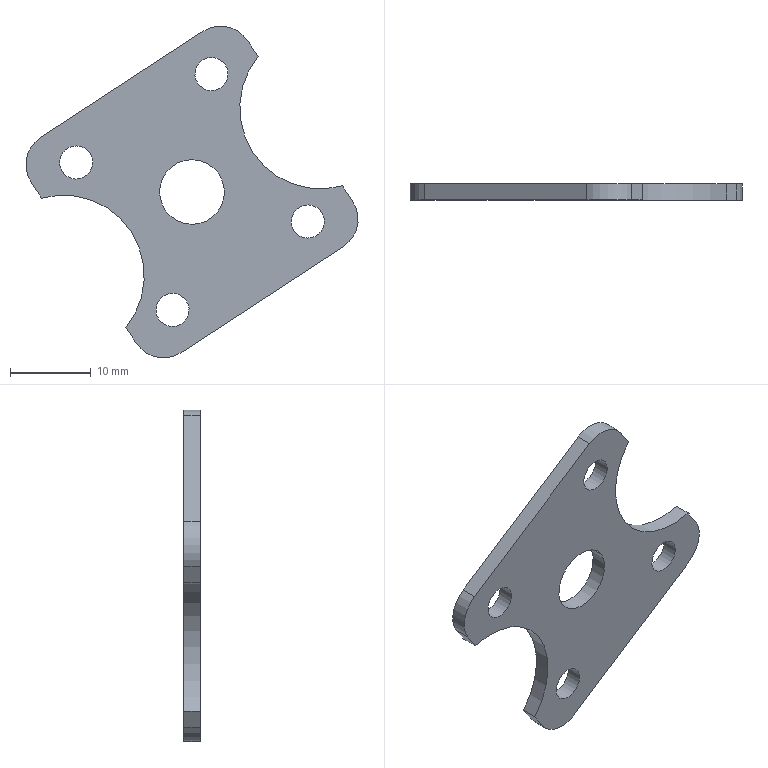Component | SolidWorks | FrontWheelSidePadPlate-1 | 1 solid | 25 faces | box 41.11 x 2 x 41.05 mm | volume 1410 mm3 | cylinder 17 | plane 8 | commonest cylinder face diameters 4.1 x8 8 x6 20 x3
build123d program:
from build123d import *

# Parameters (mm, degrees)
SKETCH1_R           = 2.05
SKETCH1_R_2         = 4
BOSS_EXTRUDE1_DEPTH = 2
FILLET1_R           = 4


with BuildPart() as part:
    # Sketch1 → Boss-Extrude1 (new body)
    with BuildSketch(Plane.XY):
        with BuildLine():
            Line((-16, -9.539), (-16, -15.9))
            Line((-16, -15.9), (16, -15.9))
            Line((16, -15.9), (16, -9.539))
            ThreePointArc((16, -9.539), (9, 0), (16, 9.539))
            Line((16, 9.539), (16, 15.9))
            Line((16, 15.9), (-16, 15.9))
            Line((-16, 15.9), (-16, 9.539))
            ThreePointArc((-16, 9.539), (-10.938, 5.916), (-9, 0))
            ThreePointArc((-9, 0), (-10.938, -5.916), (-16, -9.539))
        make_face()
        with Locations((-10, -10.9)):
            Circle(SKETCH1_R, mode=Mode.SUBTRACT)
        with Locations((10, -10.9)):
            Circle(SKETCH1_R, mode=Mode.SUBTRACT)
        with Locations((-10, 10.9)):
            Circle(SKETCH1_R, mode=Mode.SUBTRACT)
        Circle(SKETCH1_R_2, mode=Mode.SUBTRACT)
        with Locations((10, 10.9)):
            Circle(SKETCH1_R, mode=Mode.SUBTRACT)
    extrude(amount=BOSS_EXTRUDE1_DEPTH)

    # Fillet1
    fillet1_edges = [part.edges().sort_by_distance(p)[0] for p in [
        (-16, 15.9, 1),
        (16, 15.9, 1),
        (16, -15.9, 1),
        (-16, -15.9, 1),
    ]]
    fillet(fillet1_edges, radius=FILLET1_R)


solid = part.part

# Placed as in the assembly
solid = solid.moved(Location((0.3183, 28.4, 37), (90, 0, 33.158)))
STEP:
#1=CARTESIAN_POINT('',(0.175,1.118,2.075));
#2=VERTEX_POINT('',#1);
#3=CARTESIAN_POINT('',(0.03985,1.118,1.987));
#4=VERTEX_POINT('',#3);
#5=CARTESIAN_POINT('',(0.1074,1.118,2.031));
#6=DIRECTION('',(0.,-1.,0.));
#7=DIRECTION('',(0.8372,0.,0.5469));
#8=AXIS2_PLACEMENT_3D('',#5,#6,#7);
#9=CIRCLE('',#8,0.08071);
#10=EDGE_CURVE('',#2,#4,#9,.T.);
#11=ORIENTED_EDGE('',*,*,#10,.F.);
#12=CARTESIAN_POINT('',(0.175,1.039,2.075));
#13=VERTEX_POINT('',#12);
#14=CARTESIAN_POINT('',(0.175,1.118,2.075));
#15=DIRECTION('',(0.,-1.,0.));
#16=VECTOR('',#15,39.37);
#17=LINE('',#14,#16);
#18=EDGE_CURVE('',#2,#13,#17,.T.);
#19=ORIENTED_EDGE('',*,*,#18,.T.);
#20=CARTESIAN_POINT('',(0.03985,1.039,1.987));
#21=VERTEX_POINT('',#20);
#22=CARTESIAN_POINT('',(0.1074,1.039,2.031));
#23=DIRECTION('',(0.,-1.,0.));
#24=DIRECTION('',(0.8372,0.,0.5469));
#25=AXIS2_PLACEMENT_3D('',#22,#23,#24);
#26=CIRCLE('',#25,0.08071);
#27=EDGE_CURVE('',#13,#21,#26,.T.);
#28=ORIENTED_EDGE('',*,*,#27,.T.);
#29=CARTESIAN_POINT('',(0.03985,1.118,1.987));
#30=DIRECTION('',(0.,-1.,0.));
#31=VECTOR('',#30,39.37);
#32=LINE('',#29,#31);
#33=EDGE_CURVE('',#4,#21,#32,.T.);
#34=ORIENTED_EDGE('',*,*,#33,.F.);
#35=EDGE_LOOP('',(#11,#19,#28,#34));
#36=FACE_OUTER_BOUND('',#35,.T.);
#37=CARTESIAN_POINT('',(0.1074,1.118,2.031));
#38=DIRECTION('',(0.,-1.,0.));
#39=DIRECTION('',(-0.8372,0.,-0.5469));
#40=AXIS2_PLACEMENT_3D('',#37,#38,#39);
#41=CYLINDRICAL_SURFACE('',#40,0.08071);
#42=ADVANCED_FACE('',(#36),#41,.F.);
#43=CARTESIAN_POINT('',(0.5093,1.118,1.269));
#44=VERTEX_POINT('',#43);
#45=CARTESIAN_POINT('',(0.6444,1.118,1.357));
#46=VERTEX_POINT('',#45);
#47=CARTESIAN_POINT('',(0.5768,1.118,1.313));
#48=DIRECTION('',(0.,1.,0.));
#49=DIRECTION('',(0.8372,0.,0.5469));
#50=AXIS2_PLACEMENT_3D('',#47,#48,#49);
#51=CIRCLE('',#50,0.08071);
#52=EDGE_CURVE('',#44,#46,#51,.T.);
#53=ORIENTED_EDGE('',*,*,#52,.T.);
#54=CARTESIAN_POINT('',(0.6444,1.039,1.357));
#55=VERTEX_POINT('',#54);
#56=CARTESIAN_POINT('',(0.6444,1.118,1.357));
#57=DIRECTION('',(0.,-1.,0.));
#58=VECTOR('',#57,39.37);
#59=LINE('',#56,#58);
#60=EDGE_CURVE('',#46,#55,#59,.T.);
#61=ORIENTED_EDGE('',*,*,#60,.T.);
#62=CARTESIAN_POINT('',(0.5093,1.039,1.269));
#63=VERTEX_POINT('',#62);
#64=CARTESIAN_POINT('',(0.5768,1.039,1.313));
#65=DIRECTION('',(0.,1.,0.));
#66=DIRECTION('',(0.8372,0.,0.5469));
#67=AXIS2_PLACEMENT_3D('',#64,#65,#66);
#68=CIRCLE('',#67,0.08071);
#69=EDGE_CURVE('',#63,#55,#68,.T.);
#70=ORIENTED_EDGE('',*,*,#69,.F.);
#71=CARTESIAN_POINT('',(0.5093,1.118,1.269));
#72=DIRECTION('',(0.,-1.,0.));
#73=VECTOR('',#72,39.37);
#74=LINE('',#71,#73);
#75=EDGE_CURVE('',#44,#63,#74,.T.);
#76=ORIENTED_EDGE('',*,*,#75,.F.);
#77=EDGE_LOOP('',(#53,#61,#70,#76));
#78=FACE_OUTER_BOUND('',#77,.T.);
#79=CARTESIAN_POINT('',(0.5768,1.118,1.313));
#80=DIRECTION('',(0.,-1.,0.));
#81=DIRECTION('',(-0.8372,0.,-0.5469));
#82=AXIS2_PLACEMENT_3D('',#79,#80,#81);
#83=CYLINDRICAL_SURFACE('',#82,0.08071);
#84=ADVANCED_FACE('',(#78),#83,.F.);
#85=CARTESIAN_POINT('',(-0.1499,1.118,0.838));
#86=VERTEX_POINT('',#85);
#87=CARTESIAN_POINT('',(-0.01478,1.118,0.9262));
#88=VERTEX_POINT('',#87);
#89=CARTESIAN_POINT('',(-0.08235,1.118,0.8821));
#90=DIRECTION('',(0.,1.,0.));
#91=DIRECTION('',(0.8372,0.,0.5469));
#92=AXIS2_PLACEMENT_3D('',#89,#90,#91);
#93=CIRCLE('',#92,0.08071);
#94=EDGE_CURVE('',#86,#88,#93,.T.);
#95=ORIENTED_EDGE('',*,*,#94,.T.);
#96=CARTESIAN_POINT('',(-0.01478,1.039,0.9262));
#97=VERTEX_POINT('',#96);
#98=CARTESIAN_POINT('',(-0.01478,1.118,0.9262));
#99=DIRECTION('',(0.,-1.,0.));
#100=VECTOR('',#99,39.37);
#101=LINE('',#98,#100);
#102=EDGE_CURVE('',#88,#97,#101,.T.);
#103=ORIENTED_EDGE('',*,*,#102,.T.);
#104=CARTESIAN_POINT('',(-0.1499,1.039,0.838));
#105=VERTEX_POINT('',#104);
#106=CARTESIAN_POINT('',(-0.08235,1.039,0.8821));
#107=DIRECTION('',(0.,1.,0.));
#108=DIRECTION('',(0.8372,0.,0.5469));
#109=AXIS2_PLACEMENT_3D('',#106,#107,#108);
#110=CIRCLE('',#109,0.08071);
#111=EDGE_CURVE('',#105,#97,#110,.T.);
#112=ORIENTED_EDGE('',*,*,#111,.F.);
#113=CARTESIAN_POINT('',(-0.1499,1.118,0.838));
#114=DIRECTION('',(0.,-1.,0.));
#115=VECTOR('',#114,39.37);
#116=LINE('',#113,#115);
#117=EDGE_CURVE('',#86,#105,#116,.T.);
#118=ORIENTED_EDGE('',*,*,#117,.F.);
#119=EDGE_LOOP('',(#95,#103,#112,#118));
#120=FACE_OUTER_BOUND('',#119,.T.);
#121=CARTESIAN_POINT('',(-0.08235,1.118,0.8821));
#122=DIRECTION('',(0.,-1.,0.));
#123=DIRECTION('',(-0.8372,0.,-0.5469));
#124=AXIS2_PLACEMENT_3D('',#121,#122,#123);
#125=CYLINDRICAL_SURFACE('',#124,0.08071);
#126=ADVANCED_FACE('',(#120),#125,.F.);
#127=CARTESIAN_POINT('',(-0.4842,1.118,1.645));
#128=VERTEX_POINT('',#127);
#129=CARTESIAN_POINT('',(-0.6193,1.118,1.556));
#130=VERTEX_POINT('',#129);
#131=CARTESIAN_POINT('',(-0.5518,1.118,1.601));
#132=DIRECTION('',(0.,-1.,0.));
#133=DIRECTION('',(0.8372,0.,0.5469));
#134=AXIS2_PLACEMENT_3D('',#131,#132,#133);
#135=CIRCLE('',#134,0.08071);
#136=EDGE_CURVE('',#128,#130,#135,.T.);
#137=ORIENTED_EDGE('',*,*,#136,.F.);
#138=CARTESIAN_POINT('',(-0.4842,1.039,1.645));
#139=VERTEX_POINT('',#138);
#140=CARTESIAN_POINT('',(-0.4842,1.118,1.645));
#141=DIRECTION('',(0.,-1.,0.));
#142=VECTOR('',#141,39.37);
#143=LINE('',#140,#142);
#144=EDGE_CURVE('',#128,#139,#143,.T.);
#145=ORIENTED_EDGE('',*,*,#144,.T.);
#146=CARTESIAN_POINT('',(-0.6193,1.039,1.556));
#147=VERTEX_POINT('',#146);
#148=CARTESIAN_POINT('',(-0.5518,1.039,1.601));
#149=DIRECTION('',(0.,-1.,0.));
#150=DIRECTION('',(0.8372,0.,0.5469));
#151=AXIS2_PLACEMENT_3D('',#148,#149,#150);
#152=CIRCLE('',#151,0.08071);
#153=EDGE_CURVE('',#139,#147,#152,.T.);
#154=ORIENTED_EDGE('',*,*,#153,.T.);
#155=CARTESIAN_POINT('',(-0.6193,1.118,1.556));
#156=DIRECTION('',(0.,-1.,0.));
#157=VECTOR('',#156,39.37);
#158=LINE('',#155,#157);
#159=EDGE_CURVE('',#130,#147,#158,.T.);
#160=ORIENTED_EDGE('',*,*,#159,.F.);
#161=EDGE_LOOP('',(#137,#145,#154,#160));
#162=FACE_OUTER_BOUND('',#161,.T.);
#163=CARTESIAN_POINT('',(-0.5518,1.118,1.601));
#164=DIRECTION('',(0.,-1.,0.));
#165=DIRECTION('',(-0.8372,0.,-0.5469));
#166=AXIS2_PLACEMENT_3D('',#163,#164,#165);
#167=CYLINDRICAL_SURFACE('',#166,0.08071);
#168=ADVANCED_FACE('',(#162),#167,.F.);
#169=CARTESIAN_POINT('',(-0.1193,1.118,1.371));
#170=VERTEX_POINT('',#169);
#171=CARTESIAN_POINT('',(0.1444,1.118,1.543));
#172=VERTEX_POINT('',#171);
#173=CARTESIAN_POINT('',(0.01253,1.118,1.457));
#174=DIRECTION('',(0.,1.,0.));
#175=DIRECTION('',(0.8372,0.,0.5469));
#176=AXIS2_PLACEMENT_3D('',#173,#174,#175);
#177=CIRCLE('',#176,0.1575);
#178=EDGE_CURVE('',#170,#172,#177,.T.);
#179=ORIENTED_EDGE('',*,*,#178,.T.);
#180=CARTESIAN_POINT('',(0.1444,1.039,1.543));
#181=VERTEX_POINT('',#180);
#182=CARTESIAN_POINT('',(0.1444,1.118,1.543));
#183=DIRECTION('',(0.,-1.,0.));
#184=VECTOR('',#183,39.37);
#185=LINE('',#182,#184);
#186=EDGE_CURVE('',#172,#181,#185,.T.);
#187=ORIENTED_EDGE('',*,*,#186,.T.);
#188=CARTESIAN_POINT('',(-0.1193,1.039,1.371));
#189=VERTEX_POINT('',#188);
#190=CARTESIAN_POINT('',(0.01253,1.039,1.457));
#191=DIRECTION('',(0.,1.,0.));
#192=DIRECTION('',(0.8372,0.,0.5469));
#193=AXIS2_PLACEMENT_3D('',#190,#191,#192);
#194=CIRCLE('',#193,0.1575);
#195=EDGE_CURVE('',#189,#181,#194,.T.);
#196=ORIENTED_EDGE('',*,*,#195,.F.);
#197=CARTESIAN_POINT('',(-0.1193,1.118,1.371));
#198=DIRECTION('',(0.,-1.,0.));
#199=VECTOR('',#198,39.37);
#200=LINE('',#197,#199);
#201=EDGE_CURVE('',#170,#189,#200,.T.);
#202=ORIENTED_EDGE('',*,*,#201,.F.);
#203=EDGE_LOOP('',(#179,#187,#196,#202));
#204=FACE_OUTER_BOUND('',#203,.T.);
#205=CARTESIAN_POINT('',(0.01253,1.118,1.457));
#206=DIRECTION('',(0.,-1.,0.));
#207=DIRECTION('',(-0.8372,0.,-0.5469));
#208=AXIS2_PLACEMENT_3D('',#205,#206,#207);
#209=CYLINDRICAL_SURFACE('',#208,0.1575);
#210=ADVANCED_FACE('',(#204),#209,.F.);
#211=CARTESIAN_POINT('',(0.7453,1.118,1.487));
#212=VERTEX_POINT('',#211);
#213=CARTESIAN_POINT('',(0.3092,1.118,1.65));
#214=VERTEX_POINT('',#213);
#215=CARTESIAN_POINT('',(0.6388,1.118,1.866));
#216=DIRECTION('',(0.,1.,0.));
#217=DIRECTION('',(0.8372,0.,0.5469));
#218=AXIS2_PLACEMENT_3D('',#215,#216,#217);
#219=CIRCLE('',#218,0.3937);
#220=EDGE_CURVE('',#212,#214,#219,.T.);
#221=ORIENTED_EDGE('',*,*,#220,.T.);
#222=CARTESIAN_POINT('',(0.3092,1.039,1.65));
#223=VERTEX_POINT('',#222);
#224=CARTESIAN_POINT('',(0.3092,1.118,1.65));
#225=DIRECTION('',(0.,-1.,0.));
#226=VECTOR('',#225,39.37);
#227=LINE('',#224,#226);
#228=EDGE_CURVE('',#214,#223,#227,.T.);
#229=ORIENTED_EDGE('',*,*,#228,.T.);
#230=CARTESIAN_POINT('',(0.7453,1.039,1.487));
#231=VERTEX_POINT('',#230);
#232=CARTESIAN_POINT('',(0.6388,1.039,1.866));
#233=DIRECTION('',(0.,1.,0.));
#234=DIRECTION('',(0.8372,0.,0.5469));
#235=AXIS2_PLACEMENT_3D('',#232,#233,#234);
#236=CIRCLE('',#235,0.3937);
#237=EDGE_CURVE('',#231,#223,#236,.T.);
#238=ORIENTED_EDGE('',*,*,#237,.F.);
#239=CARTESIAN_POINT('',(0.7453,1.118,1.487));
#240=DIRECTION('',(0.,-1.,0.));
#241=VECTOR('',#240,39.37);
#242=LINE('',#239,#241);
#243=EDGE_CURVE('',#212,#231,#242,.T.);
#244=ORIENTED_EDGE('',*,*,#243,.F.);
#245=EDGE_LOOP('',(#221,#229,#238,#244));
#246=FACE_OUTER_BOUND('',#245,.T.);
#247=CARTESIAN_POINT('',(0.6388,1.118,1.866));
#248=DIRECTION('',(0.,-1.,0.));
#249=DIRECTION('',(-0.8372,0.,-0.5469));
#250=AXIS2_PLACEMENT_3D('',#247,#248,#249);
#251=CYLINDRICAL_SURFACE('',#250,0.3937);
#252=ADVANCED_FACE('',(#246),#251,.F.);
#253=CARTESIAN_POINT('',(-0.3094,1.118,0.7977));
#254=VERTEX_POINT('',#253);
#255=CARTESIAN_POINT('',(-0.2586,1.118,0.7199));
#256=VERTEX_POINT('',#255);
#257=CARTESIAN_POINT('',(-0.5148,1.118,1.112));
#258=DIRECTION('',(0.5469,0.,-0.8372));
#259=VECTOR('',#258,39.37);
#260=LINE('',#257,#259);
#261=EDGE_CURVE('',#254,#256,#260,.T.);
#262=ORIENTED_EDGE('',*,*,#261,.T.);
#263=CARTESIAN_POINT('',(-0.2586,1.039,0.7199));
#264=VERTEX_POINT('',#263);
#265=CARTESIAN_POINT('',(-0.2586,1.118,0.7199));
#266=DIRECTION('',(0.,-1.,0.));
#267=VECTOR('',#266,39.37);
#268=LINE('',#265,#267);
#269=EDGE_CURVE('',#256,#264,#268,.T.);
#270=ORIENTED_EDGE('',*,*,#269,.T.);
#271=CARTESIAN_POINT('',(-0.3094,1.039,0.7977));
#272=VERTEX_POINT('',#271);
#273=CARTESIAN_POINT('',(-0.5148,1.039,1.112));
#274=DIRECTION('',(0.5469,0.,-0.8372));
#275=VECTOR('',#274,39.37);
#276=LINE('',#273,#275);
#277=EDGE_CURVE('',#272,#264,#276,.T.);
#278=ORIENTED_EDGE('',*,*,#277,.F.);
#279=CARTESIAN_POINT('',(-0.3094,1.118,0.7977));
#280=DIRECTION('',(0.,-1.,0.));
#281=VECTOR('',#280,39.37);
#282=LINE('',#279,#281);
#283=EDGE_CURVE('',#254,#272,#282,.T.);
#284=ORIENTED_EDGE('',*,*,#283,.F.);
#285=EDGE_LOOP('',(#262,#270,#278,#284));
#286=FACE_OUTER_BOUND('',#285,.T.);
#287=CARTESIAN_POINT('',(-0.5148,1.118,1.112));
#288=DIRECTION('',(-0.8372,0.,-0.5469));
#289=DIRECTION('',(0.,1.,0.));
#290=AXIS2_PLACEMENT_3D('',#287,#288,#289);
#291=PLANE('',#290);
#292=ADVANCED_FACE('',(#286),#291,.T.);
#293=CARTESIAN_POINT('',(-0.7202,1.039,1.427));
#294=VERTEX_POINT('',#293);
#295=CARTESIAN_POINT('',(-0.6137,1.039,1.048));
#296=DIRECTION('',(0.,-1.,0.));
#297=DIRECTION('',(0.8372,0.,0.5469));
#298=AXIS2_PLACEMENT_3D('',#295,#296,#297);
#299=CIRCLE('',#298,0.3937);
#300=EDGE_CURVE('',#272,#294,#299,.T.);
#301=ORIENTED_EDGE('',*,*,#300,.T.);
#302=CARTESIAN_POINT('',(-0.7202,1.118,1.427));
#303=VERTEX_POINT('',#302);
#304=CARTESIAN_POINT('',(-0.7202,1.118,1.427));
#305=DIRECTION('',(0.,-1.,0.));
#306=VECTOR('',#305,39.37);
#307=LINE('',#304,#306);
#308=EDGE_CURVE('',#303,#294,#307,.T.);
#309=ORIENTED_EDGE('',*,*,#308,.F.);
#310=CARTESIAN_POINT('',(-0.6137,1.118,1.048));
#311=DIRECTION('',(0.,-1.,0.));
#312=DIRECTION('',(0.8372,0.,0.5469));
#313=AXIS2_PLACEMENT_3D('',#310,#311,#312);
#314=CIRCLE('',#313,0.3937);
#315=EDGE_CURVE('',#254,#303,#314,.T.);
#316=ORIENTED_EDGE('',*,*,#315,.F.);
#317=ORIENTED_EDGE('',*,*,#283,.T.);
#318=EDGE_LOOP('',(#301,#309,#316,#317));
#319=FACE_OUTER_BOUND('',#318,.T.);
#320=CARTESIAN_POINT('',(-0.6137,1.118,1.048));
#321=DIRECTION('',(0.,-1.,0.));
#322=DIRECTION('',(-0.8372,0.,-0.5469));
#323=AXIS2_PLACEMENT_3D('',#320,#321,#322);
#324=CYLINDRICAL_SURFACE('',#323,0.3937);
#325=ADVANCED_FACE('',(#319),#324,.F.);
#326=CARTESIAN_POINT('',(-0.7711,1.039,1.504));
#327=VERTEX_POINT('',#326);
#328=CARTESIAN_POINT('',(-0.5148,1.039,1.112));
#329=DIRECTION('',(0.5469,0.,-0.8372));
#330=VECTOR('',#329,39.37);
#331=LINE('',#328,#330);
#332=EDGE_CURVE('',#327,#294,#331,.T.);
#333=ORIENTED_EDGE('',*,*,#332,.F.);
#334=CARTESIAN_POINT('',(-0.7711,1.118,1.504));
#335=VERTEX_POINT('',#334);
#336=CARTESIAN_POINT('',(-0.7711,1.118,1.504));
#337=DIRECTION('',(0.,1.,0.));
#338=VECTOR('',#337,39.37);
#339=LINE('',#336,#338);
#340=EDGE_CURVE('',#327,#335,#339,.T.);
#341=ORIENTED_EDGE('',*,*,#340,.T.);
#342=CARTESIAN_POINT('',(-0.5148,1.118,1.112));
#343=DIRECTION('',(0.5469,0.,-0.8372));
#344=VECTOR('',#343,39.37);
#345=LINE('',#342,#344);
#346=EDGE_CURVE('',#335,#303,#345,.T.);
#347=ORIENTED_EDGE('',*,*,#346,.T.);
#348=ORIENTED_EDGE('',*,*,#308,.T.);
#349=EDGE_LOOP('',(#333,#341,#347,#348));
#350=FACE_OUTER_BOUND('',#349,.T.);
#351=CARTESIAN_POINT('',(-0.5148,1.118,1.112));
#352=DIRECTION('',(-0.8372,0.,-0.5469));
#353=DIRECTION('',(0.,1.,0.));
#354=AXIS2_PLACEMENT_3D('',#351,#352,#353);
#355=PLANE('',#354);
#356=ADVANCED_FACE('',(#350),#355,.T.);
#357=CARTESIAN_POINT('',(-0.7254,1.039,1.722));
#358=VERTEX_POINT('',#357);
#359=CARTESIAN_POINT('',(0.06567,1.039,2.239));
#360=VERTEX_POINT('',#359);
#361=CARTESIAN_POINT('',(-0.3298,1.039,1.981));
#362=DIRECTION('',(0.8372,0.,0.5469));
#363=VECTOR('',#362,39.37);
#364=LINE('',#361,#363);
#365=EDGE_CURVE('',#358,#360,#364,.T.);
#366=ORIENTED_EDGE('',*,*,#365,.T.);
#367=CARTESIAN_POINT('',(0.06567,1.118,2.239));
#368=VERTEX_POINT('',#367);
#369=CARTESIAN_POINT('',(0.06567,1.118,2.239));
#370=DIRECTION('',(0.,1.,0.));
#371=VECTOR('',#370,39.37);
#372=LINE('',#369,#371);
#373=EDGE_CURVE('',#360,#368,#372,.T.);
#374=ORIENTED_EDGE('',*,*,#373,.T.);
#375=CARTESIAN_POINT('',(-0.7254,1.118,1.722));
#376=VERTEX_POINT('',#375);
#377=CARTESIAN_POINT('',(-0.3298,1.118,1.981));
#378=DIRECTION('',(0.8372,0.,0.5469));
#379=VECTOR('',#378,39.37);
#380=LINE('',#377,#379);
#381=EDGE_CURVE('',#376,#368,#380,.T.);
#382=ORIENTED_EDGE('',*,*,#381,.F.);
#383=CARTESIAN_POINT('',(-0.7254,1.039,1.722));
#384=DIRECTION('',(0.,-1.,0.));
#385=VECTOR('',#384,39.37);
#386=LINE('',#383,#385);
#387=EDGE_CURVE('',#376,#358,#386,.T.);
#388=ORIENTED_EDGE('',*,*,#387,.T.);
#389=EDGE_LOOP('',(#366,#374,#382,#388));
#390=FACE_OUTER_BOUND('',#389,.T.);
#391=CARTESIAN_POINT('',(-0.3298,1.118,1.981));
#392=DIRECTION('',(0.5469,0.,-0.8372));
#393=DIRECTION('',(-0.8372,0.,-0.5469));
#394=AXIS2_PLACEMENT_3D('',#391,#392,#393);
#395=PLANE('',#394);
#396=ADVANCED_FACE('',(#390),#395,.F.);
#397=CARTESIAN_POINT('',(0.2836,1.118,2.193));
#398=VERTEX_POINT('',#397);
#399=CARTESIAN_POINT('',(0.3345,1.118,2.116));
#400=VERTEX_POINT('',#399);
#401=CARTESIAN_POINT('',(0.5399,1.118,1.801));
#402=DIRECTION('',(0.5469,0.,-0.8372));
#403=VECTOR('',#402,39.37);
#404=LINE('',#401,#403);
#405=EDGE_CURVE('',#398,#400,#404,.T.);
#406=ORIENTED_EDGE('',*,*,#405,.F.);
#407=CARTESIAN_POINT('',(0.2836,1.039,2.193));
#408=VERTEX_POINT('',#407);
#409=CARTESIAN_POINT('',(0.2836,1.118,2.193));
#410=DIRECTION('',(0.,-1.,0.));
#411=VECTOR('',#410,39.37);
#412=LINE('',#409,#411);
#413=EDGE_CURVE('',#398,#408,#412,.T.);
#414=ORIENTED_EDGE('',*,*,#413,.T.);
#415=CARTESIAN_POINT('',(0.3345,1.039,2.116));
#416=VERTEX_POINT('',#415);
#417=CARTESIAN_POINT('',(0.5399,1.039,1.801));
#418=DIRECTION('',(0.5469,0.,-0.8372));
#419=VECTOR('',#418,39.37);
#420=LINE('',#417,#419);
#421=EDGE_CURVE('',#408,#416,#420,.T.);
#422=ORIENTED_EDGE('',*,*,#421,.T.);
#423=CARTESIAN_POINT('',(0.3345,1.118,2.116));
#424=DIRECTION('',(0.,-1.,0.));
#425=VECTOR('',#424,39.37);
#426=LINE('',#423,#425);
#427=EDGE_CURVE('',#400,#416,#426,.T.);
#428=ORIENTED_EDGE('',*,*,#427,.F.);
#429=EDGE_LOOP('',(#406,#414,#422,#428));
#430=FACE_OUTER_BOUND('',#429,.T.);
#431=CARTESIAN_POINT('',(0.5399,1.118,1.801));
#432=DIRECTION('',(-0.8372,0.,-0.5469));
#433=DIRECTION('',(-0.5469,0.,0.8372));
#434=AXIS2_PLACEMENT_3D('',#431,#432,#433);
#435=PLANE('',#434);
#436=ADVANCED_FACE('',(#430),#435,.F.);
#437=ORIENTED_EDGE('',*,*,#228,.F.);
#438=CARTESIAN_POINT('',(0.6388,1.118,1.866));
#439=DIRECTION('',(0.,1.,0.));
#440=DIRECTION('',(0.8372,0.,0.5469));
#441=AXIS2_PLACEMENT_3D('',#438,#439,#440);
#442=CIRCLE('',#441,0.3937);
#443=EDGE_CURVE('',#214,#400,#442,.T.);
#444=ORIENTED_EDGE('',*,*,#443,.T.);
#445=ORIENTED_EDGE('',*,*,#427,.T.);
#446=CARTESIAN_POINT('',(0.6388,1.039,1.866));
#447=DIRECTION('',(0.,1.,0.));
#448=DIRECTION('',(0.8372,0.,0.5469));
#449=AXIS2_PLACEMENT_3D('',#446,#447,#448);
#450=CIRCLE('',#449,0.3937);
#451=EDGE_CURVE('',#223,#416,#450,.T.);
#452=ORIENTED_EDGE('',*,*,#451,.F.);
#453=EDGE_LOOP('',(#437,#444,#445,#452));
#454=FACE_OUTER_BOUND('',#453,.T.);
#455=CARTESIAN_POINT('',(0.6388,1.118,1.866));
#456=DIRECTION('',(0.,-1.,0.));
#457=DIRECTION('',(-0.8372,0.,-0.5469));
#458=AXIS2_PLACEMENT_3D('',#455,#456,#457);
#459=CYLINDRICAL_SURFACE('',#458,0.3937);
#460=ADVANCED_FACE('',(#454),#459,.F.);
#461=CARTESIAN_POINT('',(0.7961,1.039,1.409));
#462=VERTEX_POINT('',#461);
#463=CARTESIAN_POINT('',(0.5399,1.039,1.801));
#464=DIRECTION('',(0.5469,0.,-0.8372));
#465=VECTOR('',#464,39.37);
#466=LINE('',#463,#465);
#467=EDGE_CURVE('',#231,#462,#466,.T.);
#468=ORIENTED_EDGE('',*,*,#467,.T.);
#469=CARTESIAN_POINT('',(0.7961,1.118,1.409));
#470=VERTEX_POINT('',#469);
#471=CARTESIAN_POINT('',(0.7961,1.118,1.409));
#472=DIRECTION('',(0.,1.,0.));
#473=VECTOR('',#472,39.37);
#474=LINE('',#471,#473);
#475=EDGE_CURVE('',#462,#470,#474,.T.);
#476=ORIENTED_EDGE('',*,*,#475,.T.);
#477=CARTESIAN_POINT('',(0.5399,1.118,1.801));
#478=DIRECTION('',(0.5469,0.,-0.8372));
#479=VECTOR('',#478,39.37);
#480=LINE('',#477,#479);
#481=EDGE_CURVE('',#212,#470,#480,.T.);
#482=ORIENTED_EDGE('',*,*,#481,.F.);
#483=ORIENTED_EDGE('',*,*,#243,.T.);
#484=EDGE_LOOP('',(#468,#476,#482,#483));
#485=FACE_OUTER_BOUND('',#484,.T.);
#486=CARTESIAN_POINT('',(0.5399,1.118,1.801));
#487=DIRECTION('',(-0.8372,0.,-0.5469));
#488=DIRECTION('',(-0.5469,0.,0.8372));
#489=AXIS2_PLACEMENT_3D('',#486,#487,#488);
#490=PLANE('',#489);
#491=ADVANCED_FACE('',(#485),#490,.F.);
#492=ORIENTED_EDGE('',*,*,#186,.F.);
#493=CARTESIAN_POINT('',(0.01253,1.118,1.457));
#494=DIRECTION('',(0.,1.,0.));
#495=DIRECTION('',(0.8372,0.,0.5469));
#496=AXIS2_PLACEMENT_3D('',#493,#494,#495);
#497=CIRCLE('',#496,0.1575);
#498=EDGE_CURVE('',#172,#170,#497,.T.);
#499=ORIENTED_EDGE('',*,*,#498,.T.);
#500=ORIENTED_EDGE('',*,*,#201,.T.);
#501=CARTESIAN_POINT('',(0.01253,1.039,1.457));
#502=DIRECTION('',(0.,1.,0.));
#503=DIRECTION('',(0.8372,0.,0.5469));
#504=AXIS2_PLACEMENT_3D('',#501,#502,#503);
#505=CIRCLE('',#504,0.1575);
#506=EDGE_CURVE('',#181,#189,#505,.T.);
#507=ORIENTED_EDGE('',*,*,#506,.F.);
#508=EDGE_LOOP('',(#492,#499,#500,#507));
#509=FACE_OUTER_BOUND('',#508,.T.);
#510=CARTESIAN_POINT('',(0.01253,1.118,1.457));
#511=DIRECTION('',(0.,-1.,0.));
#512=DIRECTION('',(-0.8372,0.,-0.5469));
#513=AXIS2_PLACEMENT_3D('',#510,#511,#512);
#514=CYLINDRICAL_SURFACE('',#513,0.1575);
#515=ADVANCED_FACE('',(#509),#514,.F.);
#516=ORIENTED_EDGE('',*,*,#144,.F.);
#517=CARTESIAN_POINT('',(-0.5518,1.118,1.601));
#518=DIRECTION('',(0.,-1.,0.));
#519=DIRECTION('',(0.8372,0.,0.5469));
#520=AXIS2_PLACEMENT_3D('',#517,#518,#519);
#521=CIRCLE('',#520,0.08071);
#522=EDGE_CURVE('',#130,#128,#521,.T.);
#523=ORIENTED_EDGE('',*,*,#522,.F.);
#524=ORIENTED_EDGE('',*,*,#159,.T.);
#525=CARTESIAN_POINT('',(-0.5518,1.039,1.601));
#526=DIRECTION('',(0.,-1.,0.));
#527=DIRECTION('',(0.8372,0.,0.5469));
#528=AXIS2_PLACEMENT_3D('',#525,#526,#527);
#529=CIRCLE('',#528,0.08071);
#530=EDGE_CURVE('',#147,#139,#529,.T.);
#531=ORIENTED_EDGE('',*,*,#530,.T.);
#532=EDGE_LOOP('',(#516,#523,#524,#531));
#533=FACE_OUTER_BOUND('',#532,.T.);
#534=CARTESIAN_POINT('',(-0.5518,1.118,1.601));
#535=DIRECTION('',(0.,-1.,0.));
#536=DIRECTION('',(-0.8372,0.,-0.5469));
#537=AXIS2_PLACEMENT_3D('',#534,#535,#536);
#538=CYLINDRICAL_SURFACE('',#537,0.08071);
#539=ADVANCED_FACE('',(#533),#538,.F.);
#540=ORIENTED_EDGE('',*,*,#102,.F.);
#541=CARTESIAN_POINT('',(-0.08235,1.118,0.8821));
#542=DIRECTION('',(0.,1.,0.));
#543=DIRECTION('',(0.8372,0.,0.5469));
#544=AXIS2_PLACEMENT_3D('',#541,#542,#543);
#545=CIRCLE('',#544,0.08071);
#546=EDGE_CURVE('',#88,#86,#545,.T.);
#547=ORIENTED_EDGE('',*,*,#546,.T.);
#548=ORIENTED_EDGE('',*,*,#117,.T.);
#549=CARTESIAN_POINT('',(-0.08235,1.039,0.8821));
#550=DIRECTION('',(0.,1.,0.));
#551=DIRECTION('',(0.8372,0.,0.5469));
#552=AXIS2_PLACEMENT_3D('',#549,#550,#551);
#553=CIRCLE('',#552,0.08071);
#554=EDGE_CURVE('',#97,#105,#553,.T.);
#555=ORIENTED_EDGE('',*,*,#554,.F.);
#556=EDGE_LOOP('',(#540,#547,#548,#555));
#557=FACE_OUTER_BOUND('',#556,.T.);
#558=CARTESIAN_POINT('',(-0.08235,1.118,0.8821));
#559=DIRECTION('',(0.,-1.,0.));
#560=DIRECTION('',(-0.8372,0.,-0.5469));
#561=AXIS2_PLACEMENT_3D('',#558,#559,#560);
#562=CYLINDRICAL_SURFACE('',#561,0.08071);
#563=ADVANCED_FACE('',(#557),#562,.F.);
#564=ORIENTED_EDGE('',*,*,#60,.F.);
#565=CARTESIAN_POINT('',(0.5768,1.118,1.313));
#566=DIRECTION('',(0.,1.,0.));
#567=DIRECTION('',(0.8372,0.,0.5469));
#568=AXIS2_PLACEMENT_3D('',#565,#566,#567);
#569=CIRCLE('',#568,0.08071);
#570=EDGE_CURVE('',#46,#44,#569,.T.);
#571=ORIENTED_EDGE('',*,*,#570,.T.);
#572=ORIENTED_EDGE('',*,*,#75,.T.);
#573=CARTESIAN_POINT('',(0.5768,1.039,1.313));
#574=DIRECTION('',(0.,1.,0.));
#575=DIRECTION('',(0.8372,0.,0.5469));
#576=AXIS2_PLACEMENT_3D('',#573,#574,#575);
#577=CIRCLE('',#576,0.08071);
#578=EDGE_CURVE('',#55,#63,#577,.T.);
#579=ORIENTED_EDGE('',*,*,#578,.F.);
#580=EDGE_LOOP('',(#564,#571,#572,#579));
#581=FACE_OUTER_BOUND('',#580,.T.);
#582=CARTESIAN_POINT('',(0.5768,1.118,1.313));
#583=DIRECTION('',(0.,-1.,0.));
#584=DIRECTION('',(-0.8372,0.,-0.5469));
#585=AXIS2_PLACEMENT_3D('',#582,#583,#584);
#586=CYLINDRICAL_SURFACE('',#585,0.08071);
#587=ADVANCED_FACE('',(#581),#586,.F.);
#588=ORIENTED_EDGE('',*,*,#18,.F.);
#589=CARTESIAN_POINT('',(0.1074,1.118,2.031));
#590=DIRECTION('',(0.,-1.,0.));
#591=DIRECTION('',(0.8372,0.,0.5469));
#592=AXIS2_PLACEMENT_3D('',#589,#590,#591);
#593=CIRCLE('',#592,0.08071);
#594=EDGE_CURVE('',#4,#2,#593,.T.);
#595=ORIENTED_EDGE('',*,*,#594,.F.);
#596=ORIENTED_EDGE('',*,*,#33,.T.);
#597=CARTESIAN_POINT('',(0.1074,1.039,2.031));
#598=DIRECTION('',(0.,-1.,0.));
#599=DIRECTION('',(0.8372,0.,0.5469));
#600=AXIS2_PLACEMENT_3D('',#597,#598,#599);
#601=CIRCLE('',#600,0.08071);
#602=EDGE_CURVE('',#21,#13,#601,.T.);
#603=ORIENTED_EDGE('',*,*,#602,.T.);
#604=EDGE_LOOP('',(#588,#595,#596,#603));
#605=FACE_OUTER_BOUND('',#604,.T.);
#606=CARTESIAN_POINT('',(0.1074,1.118,2.031));
#607=DIRECTION('',(0.,-1.,0.));
#608=DIRECTION('',(-0.8372,0.,-0.5469));
#609=AXIS2_PLACEMENT_3D('',#606,#607,#608);
#610=CYLINDRICAL_SURFACE('',#609,0.08071);
#611=ADVANCED_FACE('',(#605),#610,.F.);
#612=CARTESIAN_POINT('',(-0.0406,1.118,0.6742));
#613=VERTEX_POINT('',#612);
#614=CARTESIAN_POINT('',(0.7504,1.118,1.191));
#615=VERTEX_POINT('',#614);
#616=CARTESIAN_POINT('',(0.3549,1.118,0.9326));
#617=DIRECTION('',(0.8372,0.,0.5469));
#618=VECTOR('',#617,39.37);
#619=LINE('',#616,#618);
#620=EDGE_CURVE('',#613,#615,#619,.T.);
#621=ORIENTED_EDGE('',*,*,#620,.T.);
#622=CARTESIAN_POINT('',(0.7504,1.039,1.191));
#623=VERTEX_POINT('',#622);
#624=CARTESIAN_POINT('',(0.7504,1.039,1.191));
#625=DIRECTION('',(0.,-1.,0.));
#626=VECTOR('',#625,39.37);
#627=LINE('',#624,#626);
#628=EDGE_CURVE('',#615,#623,#627,.T.);
#629=ORIENTED_EDGE('',*,*,#628,.T.);
#630=CARTESIAN_POINT('',(-0.0406,1.039,0.6742));
#631=VERTEX_POINT('',#630);
#632=CARTESIAN_POINT('',(0.3549,1.039,0.9326));
#633=DIRECTION('',(0.8372,0.,0.5469));
#634=VECTOR('',#633,39.37);
#635=LINE('',#632,#634);
#636=EDGE_CURVE('',#631,#623,#635,.T.);
#637=ORIENTED_EDGE('',*,*,#636,.F.);
#638=CARTESIAN_POINT('',(-0.0406,1.118,0.6742));
#639=DIRECTION('',(0.,1.,0.));
#640=VECTOR('',#639,39.37);
#641=LINE('',#638,#640);
#642=EDGE_CURVE('',#631,#613,#641,.T.);
#643=ORIENTED_EDGE('',*,*,#642,.T.);
#644=EDGE_LOOP('',(#621,#629,#637,#643));
#645=FACE_OUTER_BOUND('',#644,.T.);
#646=CARTESIAN_POINT('',(0.3549,1.118,0.9326));
#647=DIRECTION('',(0.5469,0.,-0.8372));
#648=DIRECTION('',(-0.8372,0.,-0.5469));
#649=AXIS2_PLACEMENT_3D('',#646,#647,#648);
#650=PLANE('',#649);
#651=ADVANCED_FACE('',(#645),#650,.T.);
#652=ORIENTED_EDGE('',*,*,#594,.T.);
#653=ORIENTED_EDGE('',*,*,#10,.T.);
#654=EDGE_LOOP('',(#652,#653));
#655=FACE_BOUND('',#654,.T.);
#656=ORIENTED_EDGE('',*,*,#52,.F.);
#657=ORIENTED_EDGE('',*,*,#570,.F.);
#658=EDGE_LOOP('',(#656,#657));
#659=FACE_BOUND('',#658,.T.);
#660=ORIENTED_EDGE('',*,*,#94,.F.);
#661=ORIENTED_EDGE('',*,*,#546,.F.);
#662=EDGE_LOOP('',(#660,#661));
#663=FACE_BOUND('',#662,.T.);
#664=ORIENTED_EDGE('',*,*,#522,.T.);
#665=ORIENTED_EDGE('',*,*,#136,.T.);
#666=EDGE_LOOP('',(#664,#665));
#667=FACE_BOUND('',#666,.T.);
#668=ORIENTED_EDGE('',*,*,#178,.F.);
#669=ORIENTED_EDGE('',*,*,#498,.F.);
#670=EDGE_LOOP('',(#668,#669));
#671=FACE_BOUND('',#670,.T.);
#672=ORIENTED_EDGE('',*,*,#381,.T.);
#673=CARTESIAN_POINT('',(0.1518,1.118,2.107));
#674=DIRECTION('',(0.,1.,0.));
#675=DIRECTION('',(0.8372,0.,0.5469));
#676=AXIS2_PLACEMENT_3D('',#673,#674,#675);
#677=CIRCLE('',#676,0.1575);
#678=EDGE_CURVE('',#368,#398,#677,.T.);
#679=ORIENTED_EDGE('',*,*,#678,.T.);
#680=ORIENTED_EDGE('',*,*,#405,.T.);
#681=ORIENTED_EDGE('',*,*,#443,.F.);
#682=ORIENTED_EDGE('',*,*,#220,.F.);
#683=ORIENTED_EDGE('',*,*,#481,.T.);
#684=CARTESIAN_POINT('',(0.6643,1.118,1.323));
#685=DIRECTION('',(0.,1.,0.));
#686=DIRECTION('',(0.8372,0.,0.5469));
#687=AXIS2_PLACEMENT_3D('',#684,#685,#686);
#688=CIRCLE('',#687,0.1575);
#689=EDGE_CURVE('',#470,#615,#688,.T.);
#690=ORIENTED_EDGE('',*,*,#689,.T.);
#691=ORIENTED_EDGE('',*,*,#620,.F.);
#692=CARTESIAN_POINT('',(-0.1267,1.118,0.8061));
#693=DIRECTION('',(0.,1.,0.));
#694=DIRECTION('',(0.8372,0.,0.5469));
#695=AXIS2_PLACEMENT_3D('',#692,#693,#694);
#696=CIRCLE('',#695,0.1575);
#697=EDGE_CURVE('',#613,#256,#696,.T.);
#698=ORIENTED_EDGE('',*,*,#697,.T.);
#699=ORIENTED_EDGE('',*,*,#261,.F.);
#700=ORIENTED_EDGE('',*,*,#315,.T.);
#701=ORIENTED_EDGE('',*,*,#346,.F.);
#702=CARTESIAN_POINT('',(-0.6392,1.118,1.591));
#703=DIRECTION('',(0.,1.,0.));
#704=DIRECTION('',(0.8372,0.,0.5469));
#705=AXIS2_PLACEMENT_3D('',#702,#703,#704);
#706=CIRCLE('',#705,0.1575);
#707=EDGE_CURVE('',#335,#376,#706,.T.);
#708=ORIENTED_EDGE('',*,*,#707,.T.);
#709=EDGE_LOOP('',(#672,#679,#680,#681,#682,#683,#690,#691,#698,#699,#700,#701,#708));
#710=FACE_OUTER_BOUND('',#709,.T.);
#711=CARTESIAN_POINT('',(0.01253,1.118,1.457));
#712=DIRECTION('',(0.,1.,0.));
#713=DIRECTION('',(0.8372,0.,0.5469));
#714=AXIS2_PLACEMENT_3D('',#711,#712,#713);
#715=PLANE('',#714);
#716=ADVANCED_FACE('',(#655,#659,#663,#667,#671,#710),#715,.T.);
#717=ORIENTED_EDGE('',*,*,#602,.F.);
#718=ORIENTED_EDGE('',*,*,#27,.F.);
#719=EDGE_LOOP('',(#717,#718));
#720=FACE_BOUND('',#719,.T.);
#721=ORIENTED_EDGE('',*,*,#69,.T.);
#722=ORIENTED_EDGE('',*,*,#578,.T.);
#723=EDGE_LOOP('',(#721,#722));
#724=FACE_BOUND('',#723,.T.);
#725=ORIENTED_EDGE('',*,*,#111,.T.);
#726=ORIENTED_EDGE('',*,*,#554,.T.);
#727=EDGE_LOOP('',(#725,#726));
#728=FACE_BOUND('',#727,.T.);
#729=ORIENTED_EDGE('',*,*,#530,.F.);
#730=ORIENTED_EDGE('',*,*,#153,.F.);
#731=EDGE_LOOP('',(#729,#730));
#732=FACE_BOUND('',#731,.T.);
#733=ORIENTED_EDGE('',*,*,#195,.T.);
#734=ORIENTED_EDGE('',*,*,#506,.T.);
#735=EDGE_LOOP('',(#733,#734));
#736=FACE_BOUND('',#735,.T.);
#737=ORIENTED_EDGE('',*,*,#421,.F.);
#738=CARTESIAN_POINT('',(0.1518,1.039,2.107));
#739=DIRECTION('',(0.,-1.,0.));
#740=DIRECTION('',(0.8372,0.,0.5469));
#741=AXIS2_PLACEMENT_3D('',#738,#739,#740);
#742=CIRCLE('',#741,0.1575);
#743=EDGE_CURVE('',#408,#360,#742,.T.);
#744=ORIENTED_EDGE('',*,*,#743,.T.);
#745=ORIENTED_EDGE('',*,*,#365,.F.);
#746=CARTESIAN_POINT('',(-0.6392,1.039,1.591));
#747=DIRECTION('',(0.,-1.,0.));
#748=DIRECTION('',(0.8372,0.,0.5469));
#749=AXIS2_PLACEMENT_3D('',#746,#747,#748);
#750=CIRCLE('',#749,0.1575);
#751=EDGE_CURVE('',#358,#327,#750,.T.);
#752=ORIENTED_EDGE('',*,*,#751,.T.);
#753=ORIENTED_EDGE('',*,*,#332,.T.);
#754=ORIENTED_EDGE('',*,*,#300,.F.);
#755=ORIENTED_EDGE('',*,*,#277,.T.);
#756=CARTESIAN_POINT('',(-0.1267,1.039,0.8061));
#757=DIRECTION('',(0.,-1.,0.));
#758=DIRECTION('',(0.8372,0.,0.5469));
#759=AXIS2_PLACEMENT_3D('',#756,#757,#758);
#760=CIRCLE('',#759,0.1575);
#761=EDGE_CURVE('',#264,#631,#760,.T.);
#762=ORIENTED_EDGE('',*,*,#761,.T.);
#763=ORIENTED_EDGE('',*,*,#636,.T.);
#764=CARTESIAN_POINT('',(0.6643,1.039,1.323));
#765=DIRECTION('',(0.,-1.,0.));
#766=DIRECTION('',(0.8372,0.,0.5469));
#767=AXIS2_PLACEMENT_3D('',#764,#765,#766);
#768=CIRCLE('',#767,0.1575);
#769=EDGE_CURVE('',#623,#462,#768,.T.);
#770=ORIENTED_EDGE('',*,*,#769,.T.);
#771=ORIENTED_EDGE('',*,*,#467,.F.);
#772=ORIENTED_EDGE('',*,*,#237,.T.);
#773=ORIENTED_EDGE('',*,*,#451,.T.);
#774=EDGE_LOOP('',(#737,#744,#745,#752,#753,#754,#755,#762,#763,#770,#771,#772,#773));
#775=FACE_OUTER_BOUND('',#774,.T.);
#776=CARTESIAN_POINT('',(0.01253,1.039,1.457));
#777=DIRECTION('',(0.,1.,0.));
#778=DIRECTION('',(0.8372,0.,0.5469));
#779=AXIS2_PLACEMENT_3D('',#776,#777,#778);
#780=PLANE('',#779);
#781=ADVANCED_FACE('',(#720,#724,#728,#732,#736,#775),#780,.F.);
#782=ORIENTED_EDGE('',*,*,#678,.F.);
#783=ORIENTED_EDGE('',*,*,#373,.F.);
#784=ORIENTED_EDGE('',*,*,#743,.F.);
#785=ORIENTED_EDGE('',*,*,#413,.F.);
#786=EDGE_LOOP('',(#782,#783,#784,#785));
#787=FACE_OUTER_BOUND('',#786,.T.);
#788=CARTESIAN_POINT('',(0.1518,1.118,2.107));
#789=DIRECTION('',(0.,-1.,0.));
#790=DIRECTION('',(-0.8372,0.,-0.5469));
#791=AXIS2_PLACEMENT_3D('',#788,#789,#790);
#792=CYLINDRICAL_SURFACE('',#791,0.1575);
#793=ADVANCED_FACE('',(#787),#792,.T.);
#794=ORIENTED_EDGE('',*,*,#707,.F.);
#795=ORIENTED_EDGE('',*,*,#340,.F.);
#796=ORIENTED_EDGE('',*,*,#751,.F.);
#797=ORIENTED_EDGE('',*,*,#387,.F.);
#798=EDGE_LOOP('',(#794,#795,#796,#797));
#799=FACE_OUTER_BOUND('',#798,.T.);
#800=CARTESIAN_POINT('',(-0.6392,1.118,1.591));
#801=DIRECTION('',(0.,1.,0.));
#802=DIRECTION('',(0.8372,0.,0.5469));
#803=AXIS2_PLACEMENT_3D('',#800,#801,#802);
#804=CYLINDRICAL_SURFACE('',#803,0.1575);
#805=ADVANCED_FACE('',(#799),#804,.T.);
#806=ORIENTED_EDGE('',*,*,#689,.F.);
#807=ORIENTED_EDGE('',*,*,#475,.F.);
#808=ORIENTED_EDGE('',*,*,#769,.F.);
#809=ORIENTED_EDGE('',*,*,#628,.F.);
#810=EDGE_LOOP('',(#806,#807,#808,#809));
#811=FACE_OUTER_BOUND('',#810,.T.);
#812=CARTESIAN_POINT('',(0.6643,1.118,1.323));
#813=DIRECTION('',(0.,1.,0.));
#814=DIRECTION('',(0.8372,0.,0.5469));
#815=AXIS2_PLACEMENT_3D('',#812,#813,#814);
#816=CYLINDRICAL_SURFACE('',#815,0.1575);
#817=ADVANCED_FACE('',(#811),#816,.T.);
#818=ORIENTED_EDGE('',*,*,#697,.F.);
#819=ORIENTED_EDGE('',*,*,#642,.F.);
#820=ORIENTED_EDGE('',*,*,#761,.F.);
#821=ORIENTED_EDGE('',*,*,#269,.F.);
#822=EDGE_LOOP('',(#818,#819,#820,#821));
#823=FACE_OUTER_BOUND('',#822,.T.);
#824=CARTESIAN_POINT('',(-0.1267,1.118,0.8061));
#825=DIRECTION('',(0.,-1.,0.));
#826=DIRECTION('',(-0.8372,0.,-0.5469));
#827=AXIS2_PLACEMENT_3D('',#824,#825,#826);
#828=CYLINDRICAL_SURFACE('',#827,0.1575);
#829=ADVANCED_FACE('',(#823),#828,.T.);
#830=CLOSED_SHELL('',(#42,#84,#126,#168,#210,#252,#292,#325,#356,#396,#436,#460,#491,#515,#539,#563,#587,#611,#651,#716,#781,#793,#805,#817,#829));
#831=MANIFOLD_SOLID_BREP('',#830);
#832=CARTESIAN_POINT('',(0.,0.,0.));
#833=DIRECTION('',(0.,0.,1.));
#834=DIRECTION('',(1.,0.,0.));
#835=AXIS2_PLACEMENT_3D('',#832,#833,#834);
#836=(LENGTH_UNIT()NAMED_UNIT(*)SI_UNIT($,.METRE.));
#837=LENGTH_MEASURE_WITH_UNIT(LENGTH_MEASURE(0.0254),#836);
#838=DIMENSIONAL_EXPONENTS(1.,0.,0.,0.,0.,0.,0.);
#839=(CONVERSION_BASED_UNIT('',#837)LENGTH_UNIT()NAMED_UNIT(#838));
#840=UNCERTAINTY_MEASURE_WITH_UNIT(LENGTH_MEASURE(0.00001),#839,'','');
#841=(NAMED_UNIT(*)PLANE_ANGLE_UNIT()SI_UNIT($,.RADIAN.));
#842=(NAMED_UNIT(*)SI_UNIT($,.STERADIAN.)SOLID_ANGLE_UNIT());
#843=(GEOMETRIC_REPRESENTATION_CONTEXT(3)GLOBAL_UNCERTAINTY_ASSIGNED_CONTEXT((#840))GLOBAL_UNIT_ASSIGNED_CONTEXT((#839,#841,#842))REPRESENTATION_CONTEXT('',''));
#844=ADVANCED_BREP_SHAPE_REPRESENTATION('',(#831,#835),#843);
#845=COLOUR_RGB('',0.7922,0.8196,0.9333);
#846=FILL_AREA_STYLE_COLOUR('',#845);
#847=FILL_AREA_STYLE('',(#846));
#848=SURFACE_STYLE_FILL_AREA(#847);
#849=SURFACE_SIDE_STYLE('',(#848));
#850=SURFACE_STYLE_USAGE(.BOTH.,#849);
#851=PRESENTATION_STYLE_ASSIGNMENT((#850));
#852=STYLED_ITEM('',(#851),#831);
#853=PRESENTATION_LAYER_ASSIGNMENT('','',(#852));
#854=(LENGTH_UNIT()NAMED_UNIT(*)SI_UNIT($,.METRE.));
#855=LENGTH_MEASURE_WITH_UNIT(LENGTH_MEASURE(0.0254),#854);
#856=DIMENSIONAL_EXPONENTS(1.,0.,0.,0.,0.,0.,0.);
#857=(CONVERSION_BASED_UNIT('',#855)LENGTH_UNIT()NAMED_UNIT(#856));
#858=UNCERTAINTY_MEASURE_WITH_UNIT(LENGTH_MEASURE(0.00001),#857,'','');
#859=(NAMED_UNIT(*)PLANE_ANGLE_UNIT()SI_UNIT($,.RADIAN.));
#860=(NAMED_UNIT(*)SI_UNIT($,.STERADIAN.)SOLID_ANGLE_UNIT());
#861=(GEOMETRIC_REPRESENTATION_CONTEXT(3)GLOBAL_UNCERTAINTY_ASSIGNED_CONTEXT((#858))GLOBAL_UNIT_ASSIGNED_CONTEXT((#857,#859,#860))REPRESENTATION_CONTEXT('',''));
#862=MECHANICAL_DESIGN_GEOMETRIC_PRESENTATION_REPRESENTATION('',(#852),#861);